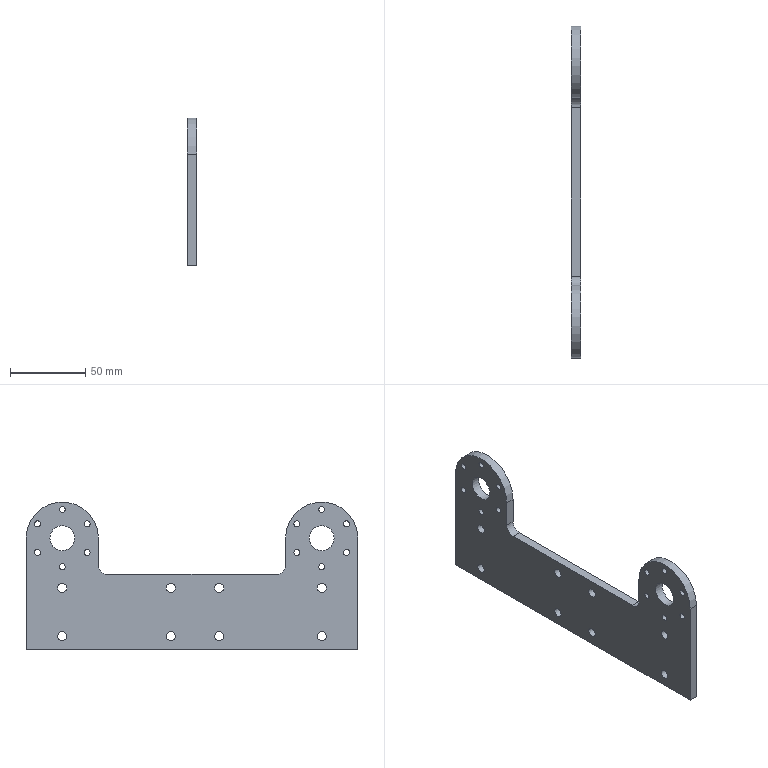Component | NX | PISTON_CYLINDER_MOUNT_PLATE | 1 solid | 34 faces | volume 85946 mm3 | cylinder 26 | plane 8 | commonest cylinder face diameters 4 x12 6 x8 48 x2 16.5 x2 12 x2